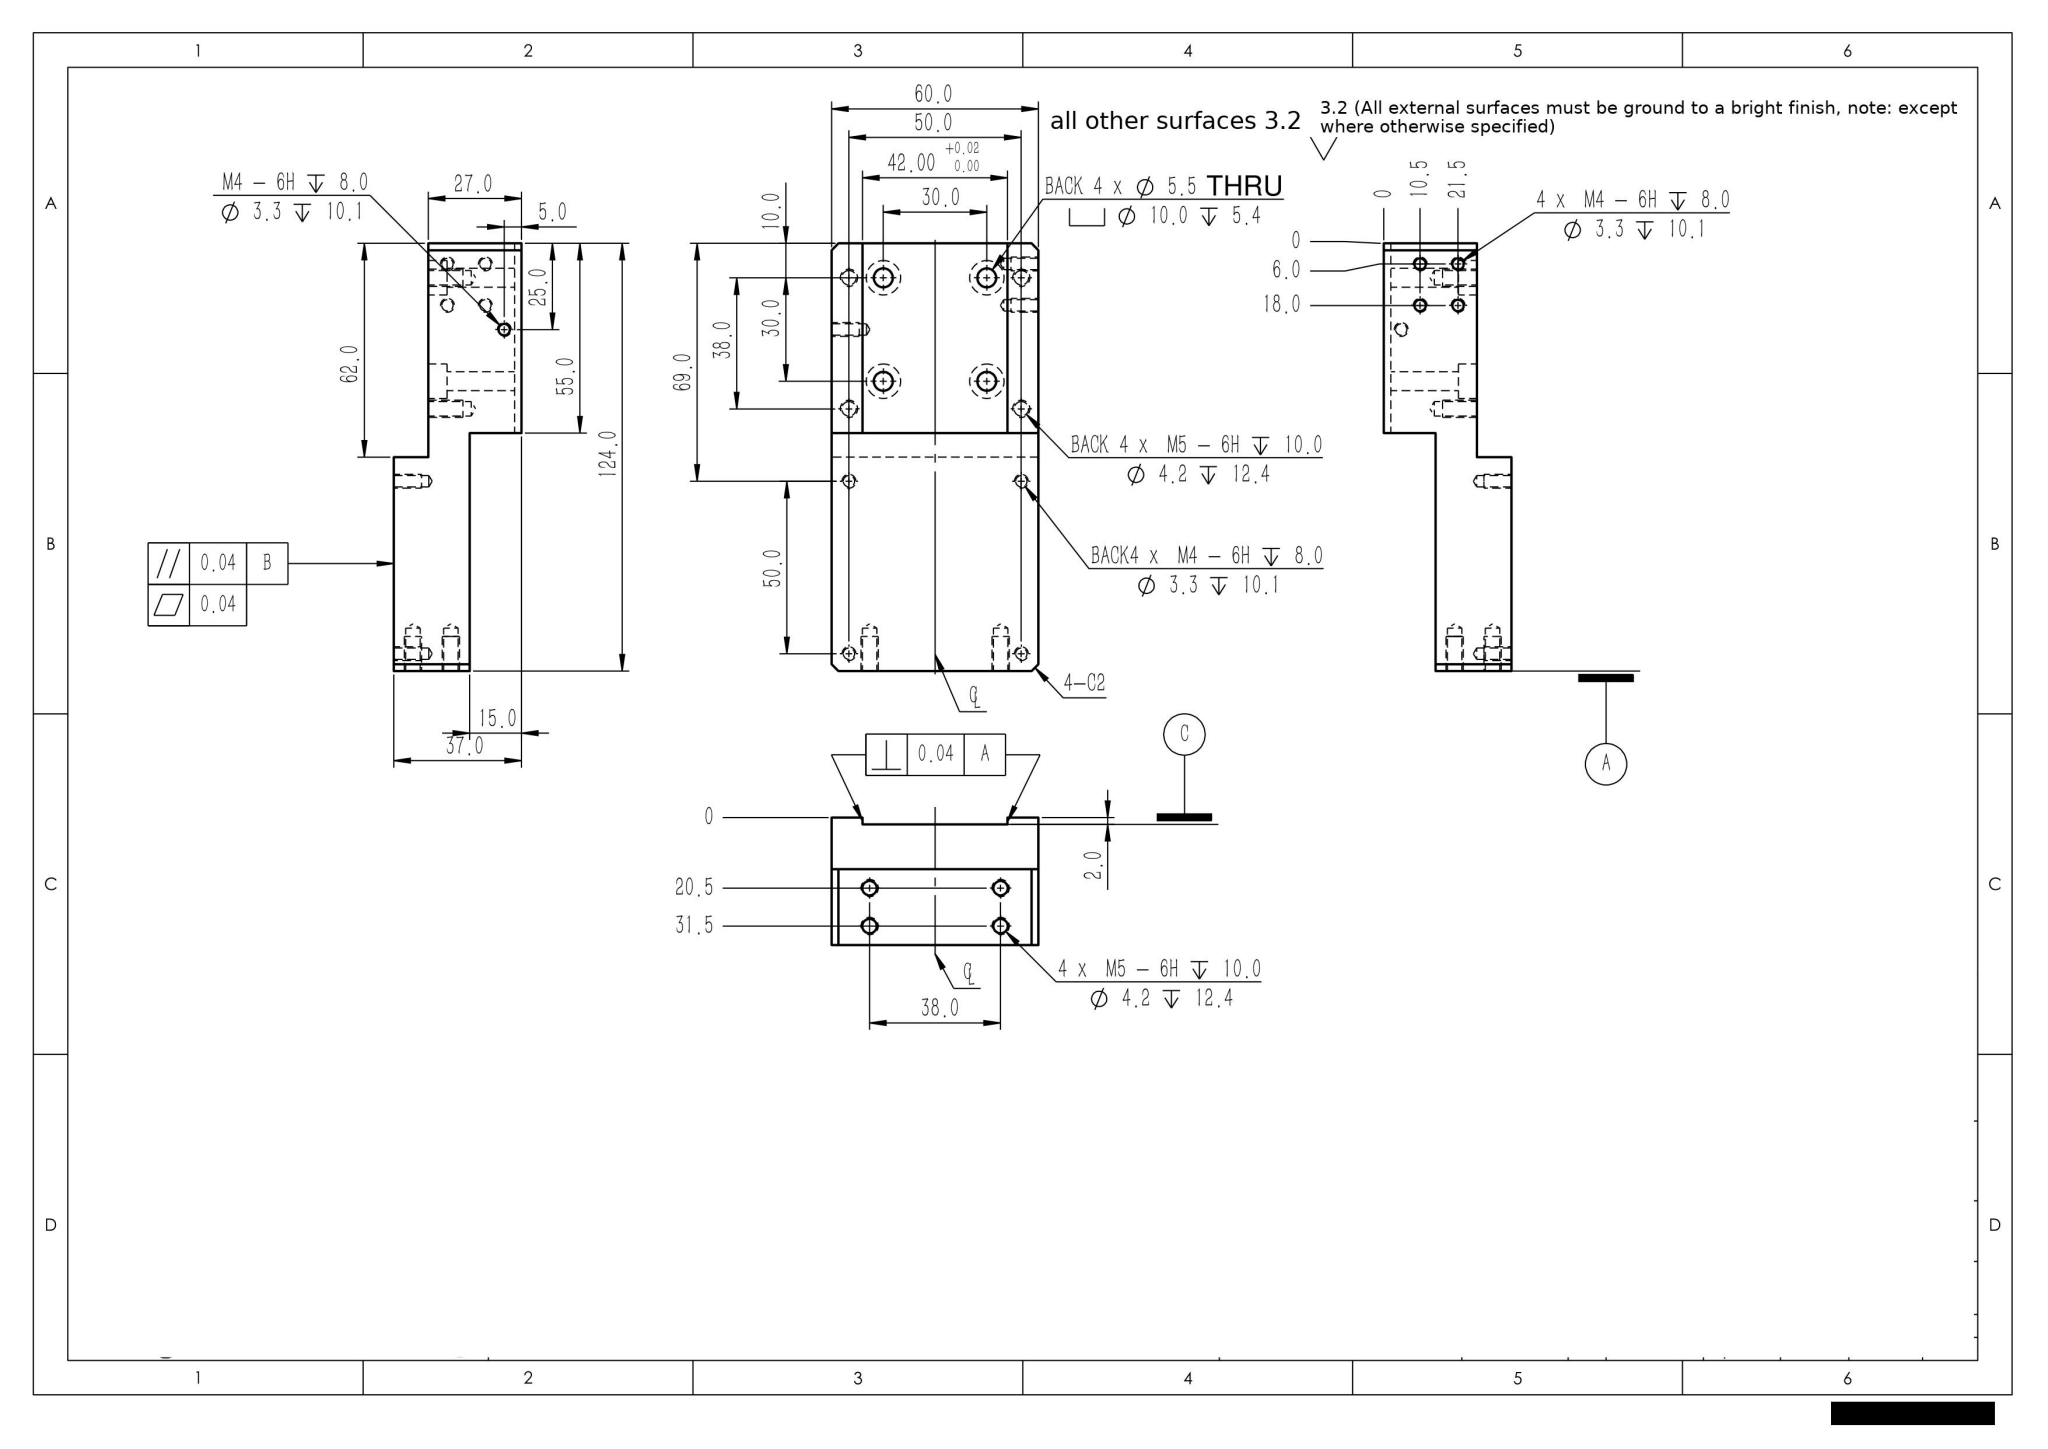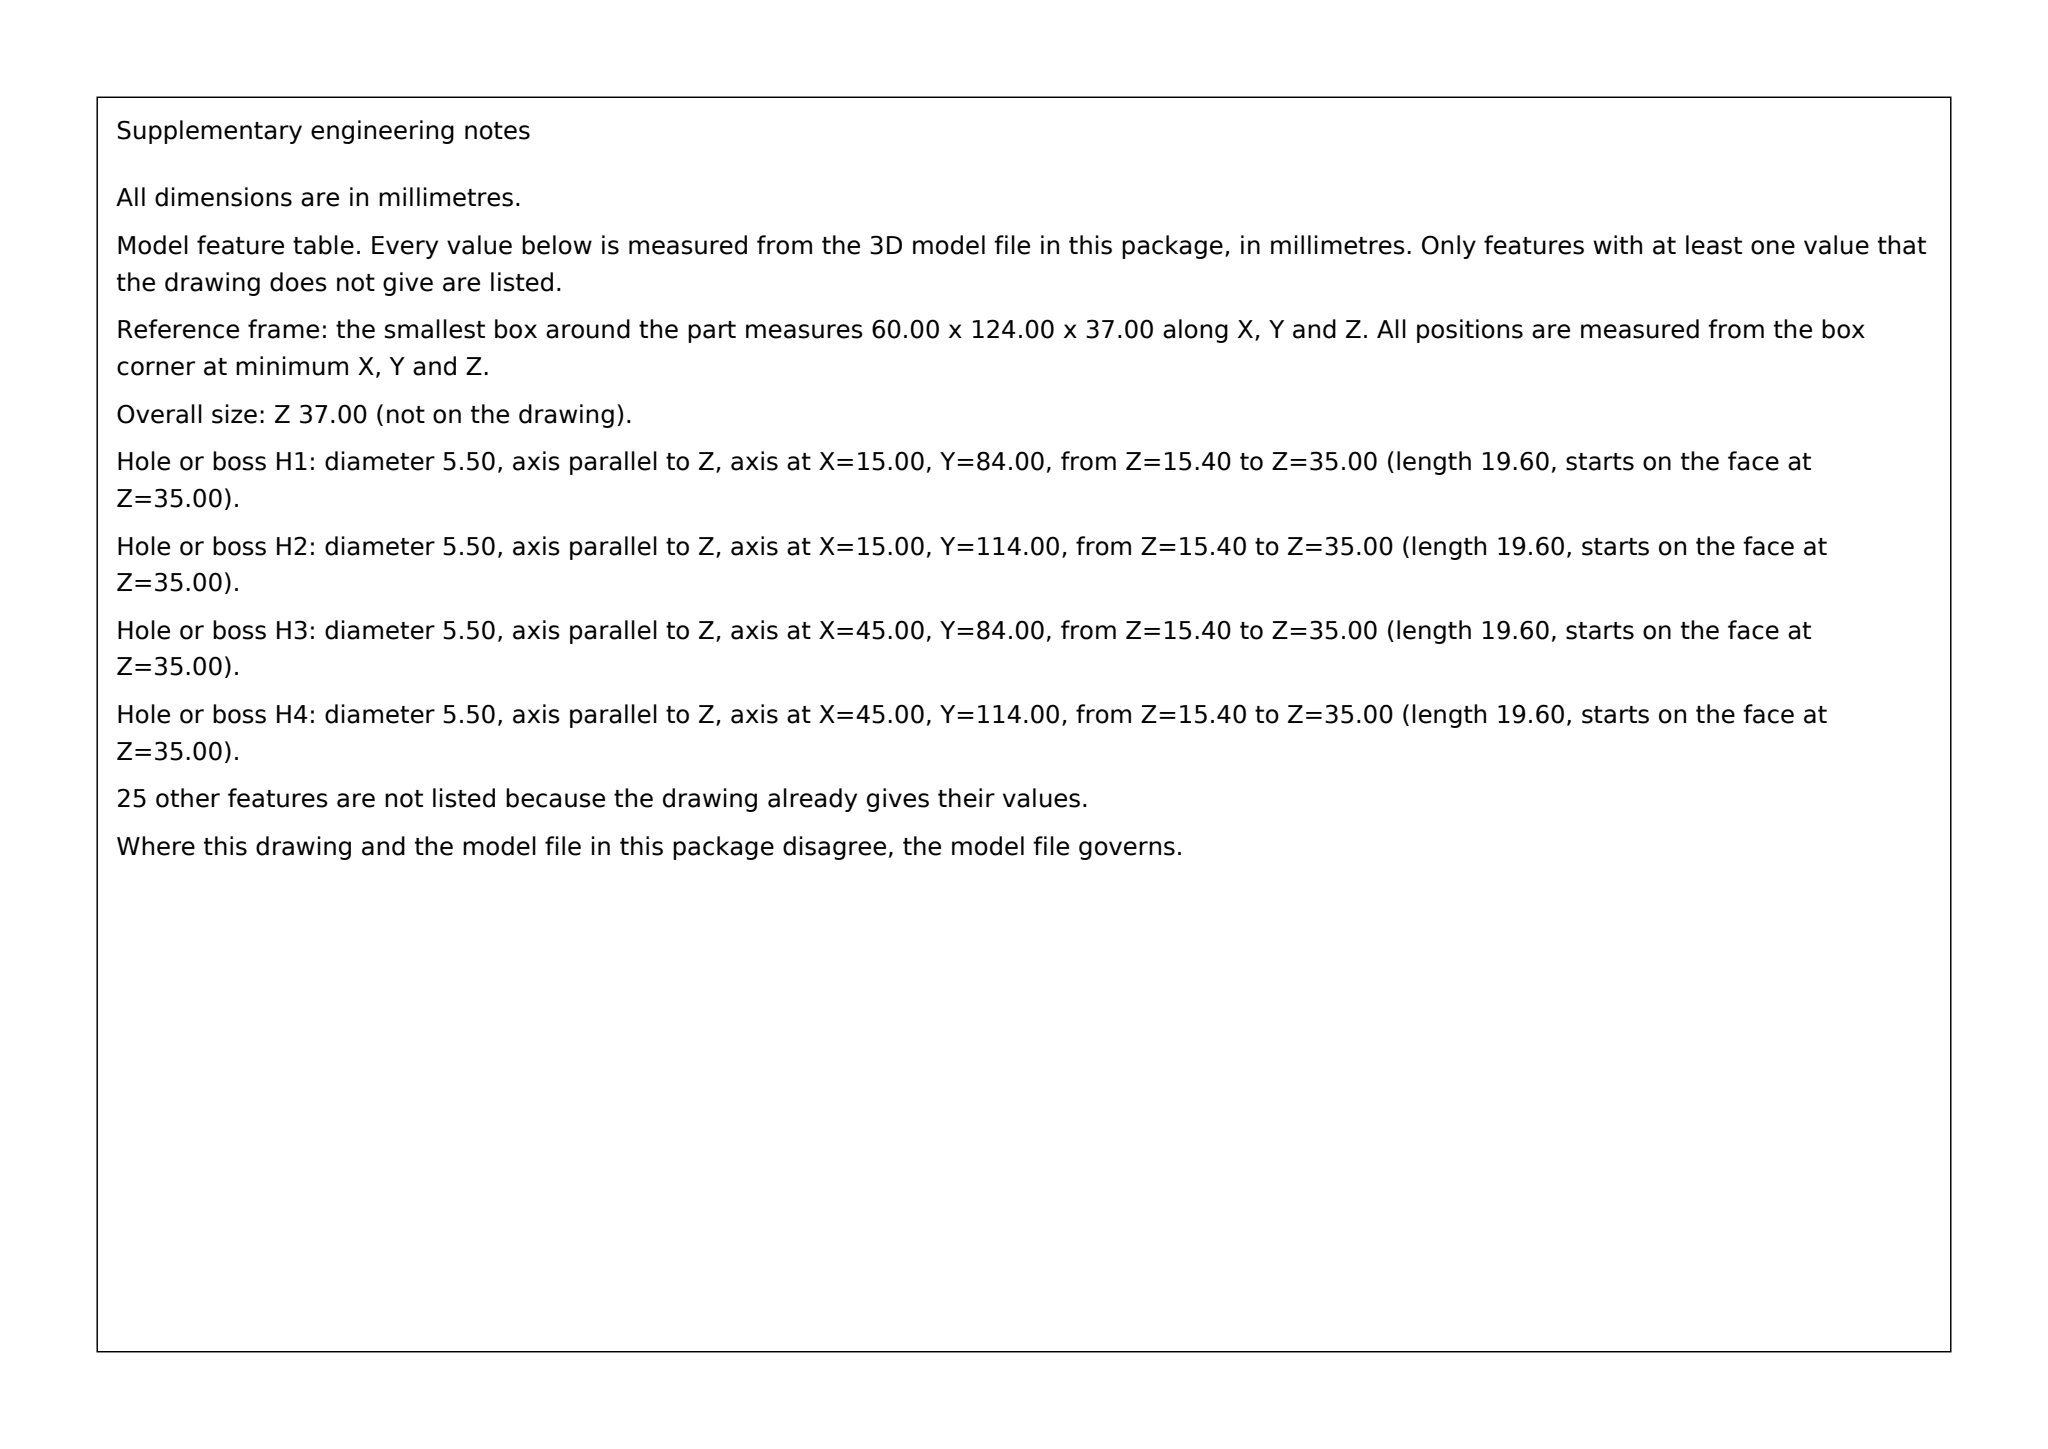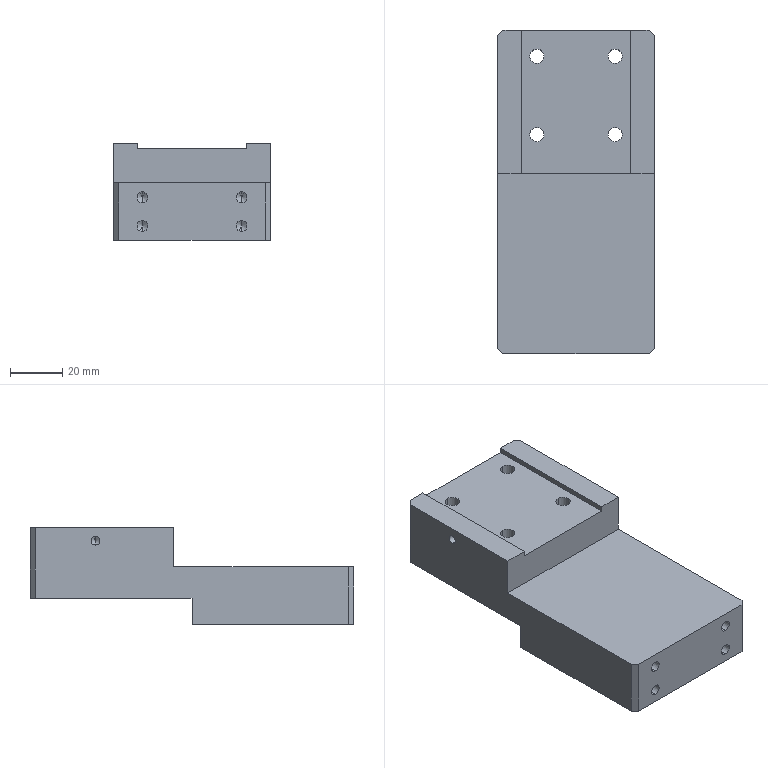Part | SolidWorks | mm | 1 solid | 106 faces | box 60 x 124 x 37 mm | volume 165381 mm3 | cylinder 50 | cone 34 | plane 22 | commonest cylinder face diameters 3.3 x18 4.2 x16 10 x8 5.5 x8
build123d program:
from build123d import *

# Parameters (mm, degrees)
SKETCH1_W                                       = 60
SKETCH1_H                                       = 124
BOSS_EXTRUDE1_DEPTH                             = 22
SKETCH2_W                                       = 60
SKETCH2_H                                       = 55
BOSS_EXTRUDE2_DEPTH                             = 15
SKETCH3_W                                       = 42
SKETCH3_H                                       = 2
CUT_EXTRUDE1_DEPTH                              = 133.834
SKETCH4_W                                       = 10
SKETCH4_H                                       = 62
CUT_EXTRUDE2_DEPTH                              = 94.878
M5_TAPPED_HOLE1_D                               = 4.2
M5_TAPPED_HOLE1_DEPTH                           = 12.4
M5_TAPPED_HOLE1_TIP                             = 1.262
M4_TAPPED_HOLE1_D                               = 3.3
M4_TAPPED_HOLE1_DEPTH                           = 10.1
M4_TAPPED_HOLE1_TIP                             = 0.9914
M5_HEX_SOCKET_HEAD_CAP_SCREW_CBORE1_D           = 5.5
M5_HEX_SOCKET_HEAD_CAP_SCREW_CBORE1_CBORE_D     = 10
M5_HEX_SOCKET_HEAD_CAP_SCREW_CBORE1_CBORE_DEPTH = 5.4
M5_TAPPED_HOLE2_D                               = 4.2
M5_TAPPED_HOLE2_DEPTH                           = 12.4
M5_TAPPED_HOLE2_TIP                             = 1.262
M4_TAPPED_HOLE2_D                               = 3.3
M4_TAPPED_HOLE2_DEPTH                           = 10.1
M4_TAPPED_HOLE2_TIP                             = 0.9914
M4_TAPPED_HOLE3_D                               = 3.3
M4_TAPPED_HOLE3_DEPTH                           = 10.1
M4_TAPPED_HOLE3_TIP                             = 0.9914
CHAMFER1_SIZE                                   = 2


with BuildPart() as part:
    # Sketch1 → Boss-Extrude1 (new body)
    with BuildSketch(Plane.XY):
        Rectangle(SKETCH1_W, SKETCH1_H)
    extrude(amount=BOSS_EXTRUDE1_DEPTH)

    # Sketch2 → Boss-Extrude2 (add)
    with BuildSketch(Plane.XY.offset(22)):
        with Locations((0, 34.5)):
            Rectangle(SKETCH2_W, SKETCH2_H)
    extrude(amount=BOSS_EXTRUDE2_DEPTH)

    # Sketch3 → Cut-Extrude1 (cut, through all)
    with BuildSketch(Plane(origin=(0, 62, 0), x_dir=(1, 0, 0), z_dir=(0, 1, 0))):
        with Locations((0, -36)):
            Rectangle(SKETCH3_W, SKETCH3_H)
    extrude(amount=-CUT_EXTRUDE1_DEPTH, mode=Mode.SUBTRACT)

    # Sketch4 → Cut-Extrude2 (cut, through all)
    with BuildSketch(Plane.ZY.offset(30)):
        with Locations((5, 31)):
            Rectangle(SKETCH4_W, SKETCH4_H)
    extrude(amount=-CUT_EXTRUDE2_DEPTH, mode=Mode.SUBTRACT)

    # M5 Tapped Hole1
    with Locations(Plane(origin=(0, -62, 0), x_dir=(-1, 0, 0), z_dir=(0, -1, 0))):
        with Locations((19, -5.5), (19, -16.5), (-19, -5.5), (-19, -16.5)):
            Hole(M5_TAPPED_HOLE1_D / 2, depth=M5_TAPPED_HOLE1_DEPTH)
            with Locations((0, 0, -(M5_TAPPED_HOLE1_DEPTH + M5_TAPPED_HOLE1_TIP / 2))):  # 118° drill point
                Cone(0, M5_TAPPED_HOLE1_D / 2, M5_TAPPED_HOLE1_TIP, mode=Mode.SUBTRACT)

    # M4 Tapped Hole1
    with Locations(Plane(origin=(0, 0, 0), x_dir=(-1, 0, 0), z_dir=(0, 0, -1))):
        with Locations((-25, -7), (25, -7), (-25, -57), (25, -57)):
            Hole(M4_TAPPED_HOLE1_D / 2, depth=M4_TAPPED_HOLE1_DEPTH)
            with Locations((0, 0, -(M4_TAPPED_HOLE1_DEPTH + M4_TAPPED_HOLE1_TIP / 2))):  # 118° drill point
                Cone(0, M4_TAPPED_HOLE1_D / 2, M4_TAPPED_HOLE1_TIP, mode=Mode.SUBTRACT)

    # M5 Hex Socket Head Cap Screw CBORE1 (through all)
    with Locations(Plane(origin=(0, 0, 10), x_dir=(-1, 0, 0), z_dir=(0, 0, -1))):
        with Locations((-15, 52), (-15, 22), (15, 22), (15, 52)):
            CounterBoreHole(M5_HEX_SOCKET_HEAD_CAP_SCREW_CBORE1_D / 2, M5_HEX_SOCKET_HEAD_CAP_SCREW_CBORE1_CBORE_D / 2, M5_HEX_SOCKET_HEAD_CAP_SCREW_CBORE1_CBORE_DEPTH)

    # M5 Tapped Hole2
    with Locations(Plane(origin=(0, 0, 10), x_dir=(-1, 0, 0), z_dir=(0, 0, -1))):
        with Locations((-25, 52), (-25, 14), (25, 14), (25, 52)):
            Hole(M5_TAPPED_HOLE2_D / 2, depth=M5_TAPPED_HOLE2_DEPTH)
            with Locations((0, 0, -(M5_TAPPED_HOLE2_DEPTH + M5_TAPPED_HOLE2_TIP / 2))):  # 118° drill point
                Cone(0, M5_TAPPED_HOLE2_D / 2, M5_TAPPED_HOLE2_TIP, mode=Mode.SUBTRACT)

    # M4 Tapped Hole2
    with Locations(Plane(origin=(30, 0, 0), x_dir=(0, 0, -1), z_dir=(1, 0, 0))):
        with Locations((-15.5, 56), (-15.5, 44), (-26.5, 56), (-26.5, 44)):
            Hole(M4_TAPPED_HOLE2_D / 2, depth=M4_TAPPED_HOLE2_DEPTH)
            with Locations((0, 0, -(M4_TAPPED_HOLE2_DEPTH + M4_TAPPED_HOLE2_TIP / 2))):  # 118° drill point
                Cone(0, M4_TAPPED_HOLE2_D / 2, M4_TAPPED_HOLE2_TIP, mode=Mode.SUBTRACT)

    # M4 Tapped Hole3
    with Locations(Plane.ZY.offset(30)):
        with Locations((32, 37)):
            Hole(M4_TAPPED_HOLE3_D / 2, depth=M4_TAPPED_HOLE3_DEPTH)
            with Locations((0, 0, -(M4_TAPPED_HOLE3_DEPTH + M4_TAPPED_HOLE3_TIP / 2))):  # 118° drill point
                Cone(0, M4_TAPPED_HOLE3_D / 2, M4_TAPPED_HOLE3_TIP, mode=Mode.SUBTRACT)

    # Chamfer1
    chamfer1_edges = [part.edges().sort_by_distance(p)[0] for p in [
        (-30, 62, 23.5),
        (30, 62, 23.5),
        (30, -62, 11),
        (-30, -62, 11),
    ]]
    chamfer(chamfer1_edges, length=CHAMFER1_SIZE)


solid = part.part